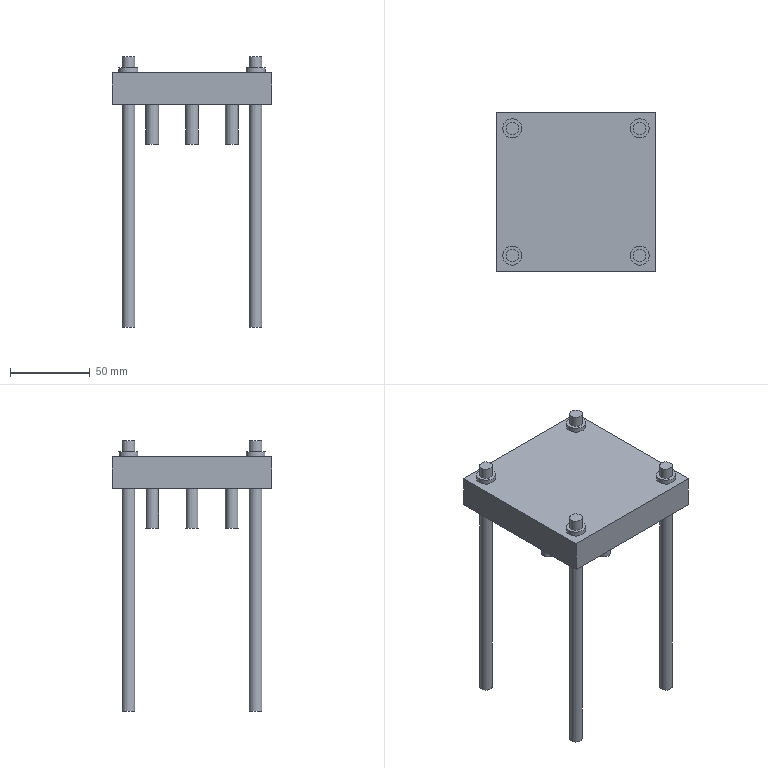Component | NX | BOLSTER | 1 solid | 48 faces | volume 232500 mm3 | plane 27 | cylinder 21 | commonest cylinder face diameters 8 x12 10 x5 12 x4